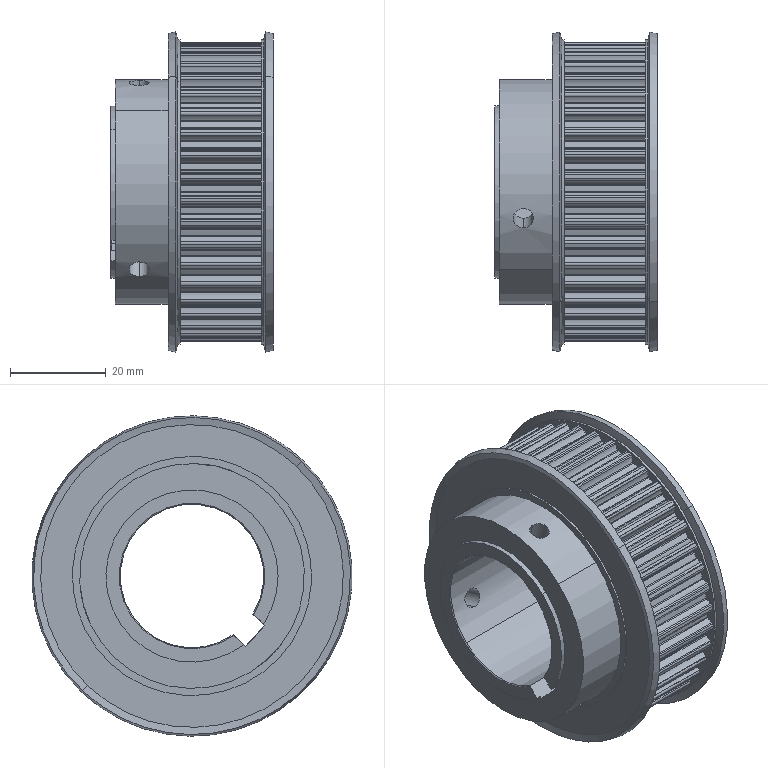Component | SolidWorks | HTPA40S5M150_B_H30-2 | 1 solid | 410 faces | box 34 x 67 x 67 mm | volume 60312 mm3 | cylinder 379 | cone 20 | plane 11 | commonest cylinder face diameters 1.1 x98 0.5 x92 6.55 x86 59.16 x41 62.7 x40 4.2 x6 50 x4 63.66 x4 | material 45#
build123d program:
from build123d import *

# Parameters (mm, degrees)
SKETCH2_W          = 127.32
SKETCH2_H          = 127.32
CUT_EXTRUDE1_DEPTH = 17
SKETCH3_W          = 6
SKETCH3_H          = 8.588
CUT_EXTRUDE2_DEPTH = 59.314
CIRPATTERN1_COUNT  = 3
SKETCH7_OUTSIDE_W  = 89.134
SKETCH7_OUTSIDE_H  = 89.134
SKETCH7_OUTSIDE_R  = 18
CUT_EXTRUDE3_DEPTH = 1


with BuildPart() as part:
    # Sketch1 → Revolve1 (revolve)
    with BuildSketch(Plane.XY, mode=Mode.PRIVATE) as revolve1_sk:
        Polygon((0, 24.8), (0, 15.2), (0.2, 15), (33.8, 15), (34, 15.2), (34, 23.3), (33.8, 23.5), (22, 23.5), (22, 25), (21.6, 25), (21.6, 31.641), (21.956, 33.127), (20.4, 33.5), (20, 31.83), (2, 31.83), (1.6, 33.5), (0.04401, 33.127), (0.4, 31.641), (0.4, 25), (0.2, 25), align=None)
    revolve(revolve1_sk.sketch.rotate(Axis((34, 0, 0), (-1, 0, 0)), 270), axis=Axis((34, 0, 0), (-1, 0, 0)))

    # Sketch2 → Cut-Extrude1 (cut)
    with BuildSketch(Plane(origin=(2.5, 0, 0), x_dir=(0, 0, -1), z_dir=(1, 0, 0))):
        Rectangle(SKETCH2_W, SKETCH2_H)
        with BuildLine():
            ThreePointArc((-31.28, 2.088), (-31.182, 1.735), (-30.884, 1.523))
            ThreePointArc((-30.884, 1.523), (-30.236, 1.259), (-29.66, 0.8639))
            ThreePointArc((-29.66, 0.8639), (-29.594, 0.7759), (-29.572, 0.6683))
            ThreePointArc((-29.572, 0.6683), (-29.58, 0), (-29.572, -0.6683))
            ThreePointArc((-29.572, -0.6683), (-29.594, -0.7759), (-29.66, -0.8639))
            ThreePointArc((-29.66, -0.8639), (-30.236, -1.259), (-30.884, -1.523))
            ThreePointArc((-30.884, -1.523), (-31.182, -1.735), (-31.28, -2.088))
            ThreePointArc((-31.28, -2.088), (-31.267, -2.274), (-31.253, -2.46))
            ThreePointArc((-31.253, -2.46), (-31.238, -2.646), (-31.222, -2.831))
            ThreePointArc((-31.222, -2.831), (-31.069, -3.164), (-30.742, -3.327))
            ThreePointArc((-30.742, -3.327), (-30.061, -3.487), (-29.43, -3.787))
            ThreePointArc((-29.43, -3.787), (-29.351, -3.863), (-29.313, -3.966))
            ThreePointArc((-29.313, -3.966), (-29.216, -4.627), (-29.104, -5.286))
            ThreePointArc((-29.104, -5.286), (-29.108, -5.396), (-29.16, -5.493))
            ThreePointArc((-29.16, -5.493), (-29.667, -5.973), (-30.265, -6.335))
            ThreePointArc((-30.265, -6.335), (-30.526, -6.592), (-30.569, -6.955))
            ThreePointArc((-30.569, -6.955), (-30.527, -7.137), (-30.484, -7.319))
            ThreePointArc((-30.484, -7.319), (-30.44, -7.5), (-30.395, -7.681))
            ThreePointArc((-30.395, -7.681), (-30.192, -7.986), (-29.843, -8.096))
            ThreePointArc((-29.843, -8.096), (-29.146, -8.146), (-28.475, -8.344))
            ThreePointArc((-28.475, -8.344), (-28.385, -8.407), (-28.332, -8.503))
            ThreePointArc((-28.332, -8.503), (-28.132, -9.141), (-27.919, -9.774))
            ThreePointArc((-27.919, -9.774), (-27.906, -9.883), (-27.941, -9.987))
            ThreePointArc((-27.941, -9.987), (-28.368, -10.541), (-28.902, -10.992))
            ThreePointArc((-28.902, -10.992), (-29.119, -11.286), (-29.104, -11.652))
            ThreePointArc((-29.104, -11.652), (-29.034, -11.825), (-28.964, -11.997))
            ThreePointArc((-28.964, -11.997), (-28.892, -12.169), (-28.819, -12.341))
            ThreePointArc((-28.819, -12.341), (-28.571, -12.61), (-28.209, -12.664))
            ThreePointArc((-28.209, -12.664), (-27.512, -12.605), (-26.819, -12.696))
            ThreePointArc((-26.819, -12.696), (-26.721, -12.744), (-26.653, -12.83))
            ThreePointArc((-26.653, -12.83), (-26.356, -13.429), (-26.046, -14.021))
            ThreePointArc((-26.046, -14.021), (-26.016, -14.127), (-26.035, -14.235))
            ThreePointArc((-26.035, -14.235), (-26.369, -14.849), (-26.826, -15.377))
            ThreePointArc((-26.826, -15.377), (-26.995, -15.702), (-26.923, -16.061))
            ThreePointArc((-26.923, -16.061), (-26.827, -16.221), (-26.73, -16.38))
            ThreePointArc((-26.73, -16.38), (-26.632, -16.539), (-26.534, -16.697))
            ThreePointArc((-26.534, -16.697), (-26.246, -16.924), (-25.88, -16.921))
            ThreePointArc((-25.88, -16.921), (-25.202, -16.754), (-24.503, -16.735))
            ThreePointArc((-24.503, -16.735), (-24.398, -16.767), (-24.317, -16.842))
            ThreePointArc((-24.317, -16.842), (-23.931, -17.387), (-23.532, -17.923))
            ThreePointArc((-23.532, -17.923), (-23.486, -18.023), (-23.488, -18.133))
            ThreePointArc((-23.488, -18.133), (-23.722, -18.791), (-24.09, -19.385))
            ThreePointArc((-24.09, -19.385), (-24.207, -19.732), (-24.079, -20.075))
            ThreePointArc((-24.079, -20.075), (-23.959, -20.218), (-23.839, -20.36))
            ThreePointArc((-23.839, -20.36), (-23.717, -20.502), (-23.595, -20.642))
            ThreePointArc((-23.595, -20.642), (-23.276, -20.822), (-22.915, -20.761))
            ThreePointArc((-22.915, -20.761), (-22.271, -20.49), (-21.584, -20.362))
            ThreePointArc((-21.584, -20.362), (-21.475, -20.378), (-21.383, -20.438))
            ThreePointArc((-21.383, -20.438), (-20.916, -20.916), (-20.438, -21.383))
            ThreePointArc((-20.438, -21.383), (-20.378, -21.475), (-20.362, -21.584))
            ThreePointArc((-20.362, -21.584), (-20.49, -22.271), (-20.761, -22.915))
            ThreePointArc((-20.761, -22.915), (-20.822, -23.276), (-20.642, -23.595))
            ThreePointArc((-20.642, -23.595), (-20.502, -23.717), (-20.36, -23.839))
            ThreePointArc((-20.36, -23.839), (-20.218, -23.959), (-20.075, -24.079))
            ThreePointArc((-20.075, -24.079), (-19.732, -24.207), (-19.385, -24.09))
            ThreePointArc((-19.385, -24.09), (-18.791, -23.722), (-18.133, -23.488))
            ThreePointArc((-18.133, -23.488), (-18.023, -23.486), (-17.923, -23.532))
            ThreePointArc((-17.923, -23.532), (-17.387, -23.931), (-16.842, -24.317))
            ThreePointArc((-16.842, -24.317), (-16.767, -24.398), (-16.735, -24.503))
            ThreePointArc((-16.735, -24.503), (-16.754, -25.202), (-16.921, -25.88))
            ThreePointArc((-16.921, -25.88), (-16.924, -26.246), (-16.697, -26.534))
            ThreePointArc((-16.697, -26.534), (-16.539, -26.632), (-16.38, -26.73))
            ThreePointArc((-16.38, -26.73), (-16.221, -26.827), (-16.061, -26.923))
            ThreePointArc((-16.061, -26.923), (-15.702, -26.995), (-15.377, -26.826))
            ThreePointArc((-15.377, -26.826), (-14.849, -26.369), (-14.235, -26.035))
            ThreePointArc((-14.235, -26.035), (-14.127, -26.016), (-14.021, -26.046))
            ThreePointArc((-14.021, -26.046), (-13.429, -26.356), (-12.83, -26.653))
            ThreePointArc((-12.83, -26.653), (-12.744, -26.721), (-12.696, -26.819))
            ThreePointArc((-12.696, -26.819), (-12.605, -27.512), (-12.664, -28.209))
            ThreePointArc((-12.664, -28.209), (-12.61, -28.571), (-12.341, -28.819))
            ThreePointArc((-12.341, -28.819), (-12.169, -28.892), (-11.997, -28.964))
            ThreePointArc((-11.997, -28.964), (-11.825, -29.034), (-11.652, -29.104))
            ThreePointArc((-11.652, -29.104), (-11.286, -29.119), (-10.992, -28.902))
            ThreePointArc((-10.992, -28.902), (-10.541, -28.368), (-9.987, -27.941))
            ThreePointArc((-9.987, -27.941), (-9.883, -27.906), (-9.774, -27.919))
            ThreePointArc((-9.774, -27.919), (-9.141, -28.132), (-8.503, -28.332))
            ThreePointArc((-8.503, -28.332), (-8.407, -28.385), (-8.344, -28.475))
            ThreePointArc((-8.344, -28.475), (-8.146, -29.146), (-8.096, -29.843))
            ThreePointArc((-8.096, -29.843), (-7.986, -30.192), (-7.681, -30.395))
            ThreePointArc((-7.681, -30.395), (-7.5, -30.44), (-7.319, -30.484))
            ThreePointArc((-7.319, -30.484), (-7.137, -30.527), (-6.955, -30.569))
            ThreePointArc((-6.955, -30.569), (-6.592, -30.526), (-6.335, -30.265))
            ThreePointArc((-6.335, -30.265), (-5.973, -29.667), (-5.493, -29.16))
            ThreePointArc((-5.493, -29.16), (-5.396, -29.108), (-5.286, -29.104))
            ThreePointArc((-5.286, -29.104), (-4.627, -29.216), (-3.966, -29.313))
            ThreePointArc((-3.966, -29.313), (-3.863, -29.351), (-3.787, -29.43))
            ThreePointArc((-3.787, -29.43), (-3.487, -30.061), (-3.327, -30.742))
            ThreePointArc((-3.327, -30.742), (-3.164, -31.069), (-2.831, -31.222))
            ThreePointArc((-2.831, -31.222), (-2.646, -31.238), (-2.46, -31.253))
            ThreePointArc((-2.46, -31.253), (-2.274, -31.267), (-2.088, -31.28))
            ThreePointArc((-2.088, -31.28), (-1.735, -31.182), (-1.523, -30.884))
            ThreePointArc((-1.523, -30.884), (-1.259, -30.236), (-0.8639, -29.66))
            ThreePointArc((-0.8639, -29.66), (-0.7759, -29.594), (-0.6683, -29.572))
            ThreePointArc((-0.6683, -29.572), (0, -29.58), (0.6683, -29.572))
            ThreePointArc((0.6683, -29.572), (0.7759, -29.594), (0.8639, -29.66))
            ThreePointArc((0.8639, -29.66), (1.259, -30.236), (1.523, -30.884))
            ThreePointArc((1.523, -30.884), (1.735, -31.182), (2.088, -31.28))
            ThreePointArc((2.088, -31.28), (2.274, -31.267), (2.46, -31.253))
            ThreePointArc((2.46, -31.253), (2.646, -31.238), (2.831, -31.222))
            ThreePointArc((2.831, -31.222), (3.164, -31.069), (3.327, -30.742))
            ThreePointArc((3.327, -30.742), (3.487, -30.061), (3.787, -29.43))
            ThreePointArc((3.787, -29.43), (3.863, -29.351), (3.966, -29.313))
            ThreePointArc((3.966, -29.313), (4.627, -29.216), (5.286, -29.104))
            ThreePointArc((5.286, -29.104), (5.396, -29.108), (5.493, -29.16))
            ThreePointArc((5.493, -29.16), (5.973, -29.667), (6.335, -30.265))
            ThreePointArc((6.335, -30.265), (6.592, -30.526), (6.955, -30.569))
            ThreePointArc((6.955, -30.569), (7.137, -30.527), (7.319, -30.484))
            ThreePointArc((7.319, -30.484), (7.5, -30.44), (7.681, -30.395))
            ThreePointArc((7.681, -30.395), (7.986, -30.192), (8.096, -29.843))
            ThreePointArc((8.096, -29.843), (8.146, -29.146), (8.344, -28.475))
            ThreePointArc((8.344, -28.475), (8.407, -28.385), (8.503, -28.332))
            ThreePointArc((8.503, -28.332), (9.141, -28.132), (9.774, -27.919))
            ThreePointArc((9.774, -27.919), (9.883, -27.906), (9.987, -27.941))
            ThreePointArc((9.987, -27.941), (10.541, -28.368), (10.992, -28.902))
            ThreePointArc((10.992, -28.902), (11.286, -29.119), (11.652, -29.104))
            ThreePointArc((11.652, -29.104), (11.825, -29.034), (11.997, -28.964))
            ThreePointArc((11.997, -28.964), (12.169, -28.892), (12.341, -28.819))
            ThreePointArc((12.341, -28.819), (12.61, -28.571), (12.664, -28.209))
            ThreePointArc((12.664, -28.209), (12.605, -27.512), (12.696, -26.819))
            ThreePointArc((12.696, -26.819), (12.744, -26.721), (12.83, -26.653))
            ThreePointArc((12.83, -26.653), (13.429, -26.356), (14.021, -26.046))
            ThreePointArc((14.021, -26.046), (14.127, -26.016), (14.235, -26.035))
            ThreePointArc((14.235, -26.035), (14.849, -26.369), (15.377, -26.826))
            ThreePointArc((15.377, -26.826), (15.702, -26.995), (16.061, -26.923))
            ThreePointArc((16.061, -26.923), (16.221, -26.827), (16.38, -26.73))
            ThreePointArc((16.38, -26.73), (16.539, -26.632), (16.697, -26.534))
            ThreePointArc((16.697, -26.534), (16.924, -26.246), (16.921, -25.88))
            ThreePointArc((16.921, -25.88), (16.754, -25.202), (16.735, -24.503))
            ThreePointArc((16.735, -24.503), (16.767, -24.398), (16.842, -24.317))
            ThreePointArc((16.842, -24.317), (17.387, -23.931), (17.923, -23.532))
            ThreePointArc((17.923, -23.532), (18.023, -23.486), (18.133, -23.488))
            ThreePointArc((18.133, -23.488), (18.791, -23.722), (19.385, -24.09))
            ThreePointArc((19.385, -24.09), (19.732, -24.207), (20.075, -24.079))
            ThreePointArc((20.075, -24.079), (20.218, -23.959), (20.36, -23.839))
            ThreePointArc((20.36, -23.839), (20.502, -23.717), (20.642, -23.595))
            ThreePointArc((20.642, -23.595), (20.822, -23.276), (20.761, -22.915))
            ThreePointArc((20.761, -22.915), (20.49, -22.271), (20.362, -21.584))
            ThreePointArc((20.362, -21.584), (20.378, -21.475), (20.438, -21.383))
            ThreePointArc((20.438, -21.383), (20.916, -20.916), (21.383, -20.438))
            ThreePointArc((21.383, -20.438), (21.475, -20.378), (21.584, -20.362))
            ThreePointArc((21.584, -20.362), (22.271, -20.49), (22.915, -20.761))
            ThreePointArc((22.915, -20.761), (23.276, -20.822), (23.595, -20.642))
            ThreePointArc((23.595, -20.642), (23.717, -20.502), (23.839, -20.36))
            ThreePointArc((23.839, -20.36), (23.959, -20.218), (24.079, -20.075))
            ThreePointArc((24.079, -20.075), (24.207, -19.732), (24.09, -19.385))
            ThreePointArc((24.09, -19.385), (23.722, -18.791), (23.488, -18.133))
            ThreePointArc((23.488, -18.133), (23.486, -18.023), (23.532, -17.923))
            ThreePointArc((23.532, -17.923), (23.931, -17.387), (24.317, -16.842))
            ThreePointArc((24.317, -16.842), (24.398, -16.767), (24.503, -16.735))
            ThreePointArc((24.503, -16.735), (25.202, -16.754), (25.88, -16.921))
            ThreePointArc((25.88, -16.921), (26.246, -16.924), (26.534, -16.697))
            ThreePointArc((26.534, -16.697), (26.632, -16.539), (26.73, -16.38))
            ThreePointArc((26.73, -16.38), (26.827, -16.221), (26.923, -16.061))
            ThreePointArc((26.923, -16.061), (26.995, -15.702), (26.826, -15.377))
            ThreePointArc((26.826, -15.377), (26.369, -14.849), (26.035, -14.235))
            ThreePointArc((26.035, -14.235), (26.016, -14.127), (26.046, -14.021))
            ThreePointArc((26.046, -14.021), (26.356, -13.429), (26.653, -12.83))
            ThreePointArc((26.653, -12.83), (26.721, -12.744), (26.819, -12.696))
            ThreePointArc((26.819, -12.696), (27.512, -12.605), (28.209, -12.664))
            ThreePointArc((28.209, -12.664), (28.571, -12.61), (28.819, -12.341))
            ThreePointArc((28.819, -12.341), (28.892, -12.169), (28.964, -11.997))
            ThreePointArc((28.964, -11.997), (29.034, -11.825), (29.104, -11.652))
            ThreePointArc((29.104, -11.652), (29.119, -11.286), (28.902, -10.992))
            ThreePointArc((28.902, -10.992), (28.368, -10.541), (27.941, -9.987))
            ThreePointArc((27.941, -9.987), (27.906, -9.883), (27.919, -9.774))
            ThreePointArc((27.919, -9.774), (28.132, -9.141), (28.332, -8.503))
            ThreePointArc((28.332, -8.503), (28.385, -8.407), (28.475, -8.344))
            ThreePointArc((28.475, -8.344), (29.146, -8.146), (29.843, -8.096))
            ThreePointArc((29.843, -8.096), (30.192, -7.986), (30.395, -7.681))
            ThreePointArc((30.395, -7.681), (30.44, -7.5), (30.484, -7.319))
            ThreePointArc((30.484, -7.319), (30.527, -7.137), (30.569, -6.955))
            ThreePointArc((30.569, -6.955), (30.526, -6.592), (30.265, -6.335))
            ThreePointArc((30.265, -6.335), (29.667, -5.973), (29.16, -5.493))
            ThreePointArc((29.16, -5.493), (29.108, -5.396), (29.104, -5.286))
            ThreePointArc((29.104, -5.286), (29.216, -4.627), (29.313, -3.966))
            ThreePointArc((29.313, -3.966), (29.351, -3.863), (29.43, -3.787))
            ThreePointArc((29.43, -3.787), (30.061, -3.487), (30.742, -3.327))
            ThreePointArc((30.742, -3.327), (31.069, -3.164), (31.222, -2.831))
            ThreePointArc((31.222, -2.831), (31.238, -2.646), (31.253, -2.46))
            ThreePointArc((31.253, -2.46), (31.267, -2.274), (31.28, -2.088))
            ThreePointArc((31.28, -2.088), (31.182, -1.735), (30.884, -1.523))
            ThreePointArc((30.884, -1.523), (30.236, -1.259), (29.66, -0.8639))
            ThreePointArc((29.66, -0.8639), (29.594, -0.7759), (29.572, -0.6683))
            ThreePointArc((29.572, -0.6683), (29.58, 0), (29.572, 0.6683))
            ThreePointArc((29.572, 0.6683), (29.594, 0.7759), (29.66, 0.8639))
            ThreePointArc((29.66, 0.8639), (30.236, 1.259), (30.884, 1.523))
            ThreePointArc((30.884, 1.523), (31.182, 1.735), (31.28, 2.088))
            ThreePointArc((31.28, 2.088), (31.267, 2.274), (31.253, 2.46))
            ThreePointArc((31.253, 2.46), (31.238, 2.646), (31.222, 2.831))
            ThreePointArc((31.222, 2.831), (31.069, 3.164), (30.742, 3.327))
            ThreePointArc((30.742, 3.327), (30.061, 3.487), (29.43, 3.787))
            ThreePointArc((29.43, 3.787), (29.351, 3.863), (29.313, 3.966))
            ThreePointArc((29.313, 3.966), (29.216, 4.627), (29.104, 5.286))
            ThreePointArc((29.104, 5.286), (29.108, 5.396), (29.16, 5.493))
            ThreePointArc((29.16, 5.493), (29.667, 5.973), (30.265, 6.335))
            ThreePointArc((30.265, 6.335), (30.526, 6.592), (30.569, 6.955))
            ThreePointArc((30.569, 6.955), (30.527, 7.137), (30.484, 7.319))
            ThreePointArc((30.484, 7.319), (30.44, 7.5), (30.395, 7.681))
            ThreePointArc((30.395, 7.681), (30.192, 7.986), (29.843, 8.096))
            ThreePointArc((29.843, 8.096), (29.146, 8.146), (28.475, 8.344))
            ThreePointArc((28.475, 8.344), (28.385, 8.407), (28.332, 8.503))
            ThreePointArc((28.332, 8.503), (28.132, 9.141), (27.919, 9.774))
            ThreePointArc((27.919, 9.774), (27.906, 9.883), (27.941, 9.987))
            ThreePointArc((27.941, 9.987), (28.368, 10.541), (28.902, 10.992))
            ThreePointArc((28.902, 10.992), (29.119, 11.286), (29.104, 11.652))
            ThreePointArc((29.104, 11.652), (29.034, 11.825), (28.964, 11.997))
            ThreePointArc((28.964, 11.997), (28.892, 12.169), (28.819, 12.341))
            ThreePointArc((28.819, 12.341), (28.571, 12.61), (28.209, 12.664))
            ThreePointArc((28.209, 12.664), (27.512, 12.605), (26.819, 12.696))
            ThreePointArc((26.819, 12.696), (26.721, 12.744), (26.653, 12.83))
            ThreePointArc((26.653, 12.83), (26.356, 13.429), (26.046, 14.021))
            ThreePointArc((26.046, 14.021), (26.016, 14.127), (26.035, 14.235))
            ThreePointArc((26.035, 14.235), (26.369, 14.849), (26.826, 15.377))
            ThreePointArc((26.826, 15.377), (26.995, 15.702), (26.923, 16.061))
            ThreePointArc((26.923, 16.061), (26.827, 16.221), (26.73, 16.38))
            ThreePointArc((26.73, 16.38), (26.632, 16.539), (26.534, 16.697))
            ThreePointArc((26.534, 16.697), (26.246, 16.924), (25.88, 16.921))
            ThreePointArc((25.88, 16.921), (25.202, 16.754), (24.503, 16.735))
            ThreePointArc((24.503, 16.735), (24.398, 16.767), (24.317, 16.842))
            ThreePointArc((24.317, 16.842), (23.931, 17.387), (23.532, 17.923))
            ThreePointArc((23.532, 17.923), (23.486, 18.023), (23.488, 18.133))
            ThreePointArc((23.488, 18.133), (23.722, 18.791), (24.09, 19.385))
            ThreePointArc((24.09, 19.385), (24.207, 19.732), (24.079, 20.075))
            ThreePointArc((24.079, 20.075), (23.959, 20.218), (23.839, 20.36))
            ThreePointArc((23.839, 20.36), (23.717, 20.502), (23.595, 20.642))
            ThreePointArc((23.595, 20.642), (23.276, 20.822), (22.915, 20.761))
            ThreePointArc((22.915, 20.761), (22.271, 20.49), (21.584, 20.362))
            ThreePointArc((21.584, 20.362), (21.475, 20.378), (21.383, 20.438))
            ThreePointArc((21.383, 20.438), (20.916, 20.916), (20.438, 21.383))
            ThreePointArc((20.438, 21.383), (20.378, 21.475), (20.362, 21.584))
            ThreePointArc((20.362, 21.584), (20.49, 22.271), (20.761, 22.915))
            ThreePointArc((20.761, 22.915), (20.822, 23.276), (20.642, 23.595))
            ThreePointArc((20.642, 23.595), (20.502, 23.717), (20.36, 23.839))
            ThreePointArc((20.36, 23.839), (20.218, 23.959), (20.075, 24.079))
            ThreePointArc((20.075, 24.079), (19.732, 24.207), (19.385, 24.09))
            ThreePointArc((19.385, 24.09), (18.791, 23.722), (18.133, 23.488))
            ThreePointArc((18.133, 23.488), (18.023, 23.486), (17.923, 23.532))
            ThreePointArc((17.923, 23.532), (17.387, 23.931), (16.842, 24.317))
            ThreePointArc((16.842, 24.317), (16.767, 24.398), (16.735, 24.503))
            ThreePointArc((16.735, 24.503), (16.754, 25.202), (16.921, 25.88))
            ThreePointArc((16.921, 25.88), (16.924, 26.246), (16.697, 26.534))
            ThreePointArc((16.697, 26.534), (16.539, 26.632), (16.38, 26.73))
            ThreePointArc((16.38, 26.73), (16.221, 26.827), (16.061, 26.923))
            ThreePointArc((16.061, 26.923), (15.702, 26.995), (15.377, 26.826))
            ThreePointArc((15.377, 26.826), (14.849, 26.369), (14.235, 26.035))
            ThreePointArc((14.235, 26.035), (14.127, 26.016), (14.021, 26.046))
            ThreePointArc((14.021, 26.046), (13.429, 26.356), (12.83, 26.653))
            ThreePointArc((12.83, 26.653), (12.744, 26.721), (12.696, 26.819))
            ThreePointArc((12.696, 26.819), (12.605, 27.512), (12.664, 28.209))
            ThreePointArc((12.664, 28.209), (12.61, 28.571), (12.341, 28.819))
            ThreePointArc((12.341, 28.819), (12.169, 28.892), (11.997, 28.964))
            ThreePointArc((11.997, 28.964), (11.825, 29.034), (11.652, 29.104))
            ThreePointArc((11.652, 29.104), (11.286, 29.119), (10.992, 28.902))
            ThreePointArc((10.992, 28.902), (10.541, 28.368), (9.987, 27.941))
            ThreePointArc((9.987, 27.941), (9.883, 27.906), (9.774, 27.919))
            ThreePointArc((9.774, 27.919), (9.141, 28.132), (8.503, 28.332))
            ThreePointArc((8.503, 28.332), (8.407, 28.385), (8.344, 28.475))
            ThreePointArc((8.344, 28.475), (8.146, 29.146), (8.096, 29.843))
            ThreePointArc((8.096, 29.843), (7.986, 30.192), (7.681, 30.395))
            ThreePointArc((7.681, 30.395), (7.5, 30.44), (7.319, 30.484))
            ThreePointArc((7.319, 30.484), (7.137, 30.527), (6.955, 30.569))
            ThreePointArc((6.955, 30.569), (6.592, 30.526), (6.335, 30.265))
            ThreePointArc((6.335, 30.265), (5.973, 29.667), (5.493, 29.16))
            ThreePointArc((5.493, 29.16), (5.396, 29.108), (5.286, 29.104))
            ThreePointArc((5.286, 29.104), (4.627, 29.216), (3.966, 29.313))
            ThreePointArc((3.966, 29.313), (3.863, 29.351), (3.787, 29.43))
            ThreePointArc((3.787, 29.43), (3.487, 30.061), (3.327, 30.742))
            ThreePointArc((3.327, 30.742), (3.164, 31.069), (2.831, 31.222))
            ThreePointArc((2.831, 31.222), (2.646, 31.238), (2.46, 31.253))
            ThreePointArc((2.46, 31.253), (2.274, 31.267), (2.088, 31.28))
            ThreePointArc((2.088, 31.28), (1.735, 31.182), (1.523, 30.884))
            ThreePointArc((1.523, 30.884), (1.259, 30.236), (0.8639, 29.66))
            ThreePointArc((0.8639, 29.66), (0.7759, 29.594), (0.6683, 29.572))
            ThreePointArc((0.6683, 29.572), (0, 29.58), (-0.6683, 29.572))
            ThreePointArc((-0.6683, 29.572), (-0.7759, 29.594), (-0.8639, 29.66))
            ThreePointArc((-0.8639, 29.66), (-1.259, 30.236), (-1.523, 30.884))
            ThreePointArc((-1.523, 30.884), (-1.735, 31.182), (-2.088, 31.28))
            ThreePointArc((-2.088, 31.28), (-2.274, 31.267), (-2.46, 31.253))
            ThreePointArc((-2.46, 31.253), (-2.646, 31.238), (-2.831, 31.222))
            ThreePointArc((-2.831, 31.222), (-3.164, 31.069), (-3.327, 30.742))
            ThreePointArc((-3.327, 30.742), (-3.487, 30.061), (-3.787, 29.43))
            ThreePointArc((-3.787, 29.43), (-3.863, 29.351), (-3.966, 29.313))
            ThreePointArc((-3.966, 29.313), (-4.627, 29.216), (-5.286, 29.104))
            ThreePointArc((-5.286, 29.104), (-5.396, 29.108), (-5.493, 29.16))
            ThreePointArc((-5.493, 29.16), (-5.973, 29.667), (-6.335, 30.265))
            ThreePointArc((-6.335, 30.265), (-6.592, 30.526), (-6.955, 30.569))
            ThreePointArc((-6.955, 30.569), (-7.137, 30.527), (-7.319, 30.484))
            ThreePointArc((-7.319, 30.484), (-7.5, 30.44), (-7.681, 30.395))
            ThreePointArc((-7.681, 30.395), (-7.986, 30.192), (-8.096, 29.843))
            ThreePointArc((-8.096, 29.843), (-8.146, 29.146), (-8.344, 28.475))
            ThreePointArc((-8.344, 28.475), (-8.407, 28.385), (-8.503, 28.332))
            ThreePointArc((-8.503, 28.332), (-9.141, 28.132), (-9.774, 27.919))
            ThreePointArc((-9.774, 27.919), (-9.883, 27.906), (-9.987, 27.941))
            ThreePointArc((-9.987, 27.941), (-10.541, 28.368), (-10.992, 28.902))
            ThreePointArc((-10.992, 28.902), (-11.286, 29.119), (-11.652, 29.104))
            ThreePointArc((-11.652, 29.104), (-11.825, 29.034), (-11.997, 28.964))
            ThreePointArc((-11.997, 28.964), (-12.169, 28.892), (-12.341, 28.819))
            ThreePointArc((-12.341, 28.819), (-12.61, 28.571), (-12.664, 28.209))
            ThreePointArc((-12.664, 28.209), (-12.605, 27.512), (-12.696, 26.819))
            ThreePointArc((-12.696, 26.819), (-12.744, 26.721), (-12.83, 26.653))
            ThreePointArc((-12.83, 26.653), (-13.429, 26.356), (-14.021, 26.046))
            ThreePointArc((-14.021, 26.046), (-14.127, 26.016), (-14.235, 26.035))
            ThreePointArc((-14.235, 26.035), (-14.849, 26.369), (-15.377, 26.826))
            ThreePointArc((-15.377, 26.826), (-15.702, 26.995), (-16.061, 26.923))
            ThreePointArc((-16.061, 26.923), (-16.221, 26.827), (-16.38, 26.73))
            ThreePointArc((-16.38, 26.73), (-16.539, 26.632), (-16.697, 26.534))
            ThreePointArc((-16.697, 26.534), (-16.924, 26.246), (-16.921, 25.88))
            ThreePointArc((-16.921, 25.88), (-16.754, 25.202), (-16.735, 24.503))
            ThreePointArc((-16.735, 24.503), (-16.767, 24.398), (-16.842, 24.317))
            ThreePointArc((-16.842, 24.317), (-17.387, 23.931), (-17.923, 23.532))
            ThreePointArc((-17.923, 23.532), (-18.023, 23.486), (-18.133, 23.488))
            ThreePointArc((-18.133, 23.488), (-18.791, 23.722), (-19.385, 24.09))
            ThreePointArc((-19.385, 24.09), (-19.732, 24.207), (-20.075, 24.079))
            ThreePointArc((-20.075, 24.079), (-20.218, 23.959), (-20.36, 23.839))
            ThreePointArc((-20.36, 23.839), (-20.502, 23.717), (-20.642, 23.595))
            ThreePointArc((-20.642, 23.595), (-20.822, 23.276), (-20.761, 22.915))
            ThreePointArc((-20.761, 22.915), (-20.49, 22.271), (-20.362, 21.584))
            ThreePointArc((-20.362, 21.584), (-20.378, 21.475), (-20.438, 21.383))
            ThreePointArc((-20.438, 21.383), (-20.916, 20.916), (-21.383, 20.438))
            ThreePointArc((-21.383, 20.438), (-21.475, 20.378), (-21.584, 20.362))
            ThreePointArc((-21.584, 20.362), (-22.271, 20.49), (-22.915, 20.761))
            ThreePointArc((-22.915, 20.761), (-23.276, 20.822), (-23.595, 20.642))
            ThreePointArc((-23.595, 20.642), (-23.717, 20.502), (-23.839, 20.36))
            ThreePointArc((-23.839, 20.36), (-23.959, 20.218), (-24.079, 20.075))
            ThreePointArc((-24.079, 20.075), (-24.207, 19.732), (-24.09, 19.385))
            ThreePointArc((-24.09, 19.385), (-23.722, 18.791), (-23.488, 18.133))
            ThreePointArc((-23.488, 18.133), (-23.486, 18.023), (-23.532, 17.923))
            ThreePointArc((-23.532, 17.923), (-23.931, 17.387), (-24.317, 16.842))
            ThreePointArc((-24.317, 16.842), (-24.398, 16.767), (-24.503, 16.735))
            ThreePointArc((-24.503, 16.735), (-25.202, 16.754), (-25.88, 16.921))
            ThreePointArc((-25.88, 16.921), (-26.246, 16.924), (-26.534, 16.697))
            ThreePointArc((-26.534, 16.697), (-26.632, 16.539), (-26.73, 16.38))
            ThreePointArc((-26.73, 16.38), (-26.827, 16.221), (-26.923, 16.061))
            ThreePointArc((-26.923, 16.061), (-26.995, 15.702), (-26.826, 15.377))
            ThreePointArc((-26.826, 15.377), (-26.369, 14.849), (-26.035, 14.235))
            ThreePointArc((-26.035, 14.235), (-26.016, 14.127), (-26.046, 14.021))
            ThreePointArc((-26.046, 14.021), (-26.356, 13.429), (-26.653, 12.83))
            ThreePointArc((-26.653, 12.83), (-26.721, 12.744), (-26.819, 12.696))
            ThreePointArc((-26.819, 12.696), (-27.512, 12.605), (-28.209, 12.664))
            ThreePointArc((-28.209, 12.664), (-28.571, 12.61), (-28.819, 12.341))
            ThreePointArc((-28.819, 12.341), (-28.892, 12.169), (-28.964, 11.997))
            ThreePointArc((-28.964, 11.997), (-29.034, 11.825), (-29.104, 11.652))
            ThreePointArc((-29.104, 11.652), (-29.119, 11.286), (-28.902, 10.992))
            ThreePointArc((-28.902, 10.992), (-28.368, 10.541), (-27.941, 9.987))
            ThreePointArc((-27.941, 9.987), (-27.906, 9.883), (-27.919, 9.774))
            ThreePointArc((-27.919, 9.774), (-28.132, 9.141), (-28.332, 8.503))
            ThreePointArc((-28.332, 8.503), (-28.385, 8.407), (-28.475, 8.344))
            ThreePointArc((-28.475, 8.344), (-29.146, 8.146), (-29.843, 8.096))
            ThreePointArc((-29.843, 8.096), (-30.192, 7.986), (-30.395, 7.681))
            ThreePointArc((-30.395, 7.681), (-30.44, 7.5), (-30.484, 7.319))
            ThreePointArc((-30.484, 7.319), (-30.527, 7.137), (-30.569, 6.955))
            ThreePointArc((-30.569, 6.955), (-30.526, 6.592), (-30.265, 6.335))
            ThreePointArc((-30.265, 6.335), (-29.667, 5.973), (-29.16, 5.493))
            ThreePointArc((-29.16, 5.493), (-29.108, 5.396), (-29.104, 5.286))
            ThreePointArc((-29.104, 5.286), (-29.216, 4.627), (-29.313, 3.966))
            ThreePointArc((-29.313, 3.966), (-29.351, 3.863), (-29.43, 3.787))
            ThreePointArc((-29.43, 3.787), (-30.061, 3.487), (-30.742, 3.327))
            ThreePointArc((-30.742, 3.327), (-31.069, 3.164), (-31.222, 2.831))
            ThreePointArc((-31.222, 2.831), (-31.238, 2.646), (-31.253, 2.46))
            ThreePointArc((-31.253, 2.46), (-31.267, 2.274), (-31.28, 2.088))
        make_face(mode=Mode.SUBTRACT)
    extrude(amount=CUT_EXTRUDE1_DEPTH, mode=Mode.SUBTRACT)

    # Sketch3 → Cut-Extrude2 (cut, through all)
    with BuildSketch(Plane(origin=(34, 0, 0), x_dir=(0, 0, -1), z_dir=(1, 0, 0))):
        with Locations((0, 13.906)):
            Rectangle(SKETCH3_W, SKETCH3_H)
    extrude(amount=-CUT_EXTRUDE2_DEPTH, mode=Mode.SUBTRACT)

    # Sketch6 → M5 Tapped Hole1 (revolve, cut)
    with BuildSketch(Plane(origin=(28, 0, 0), x_dir=(0, 0, -1), z_dir=(1, 0, 0))):
        Polygon((0, 0), (0, 45.762), (2.1, 45.762), (2.1, 0.425), (2.525, 0), align=None)
    m5_tapped_hole1 = revolve(axis=Axis((28, -6.35, 0), (0, 1, 0)), mode=Mode.SUBTRACT)

    # CirPattern1: M5 Tapped Hole1 ×3 about axis
    cirpattern1_axis = Axis((33.8, 0, 0), (-1, 0, 0))
    for i in range(1, CIRPATTERN1_COUNT):
        add(m5_tapped_hole1.rotate(cirpattern1_axis, i * 360 / CIRPATTERN1_COUNT), mode=Mode.SUBTRACT)

    # Sketch7 outside → Cut-Extrude3 (cut)
    with BuildSketch(Plane(origin=(34, 0, 0), x_dir=(0, 0, -1), z_dir=(1, 0, 0))):
        Rectangle(SKETCH7_OUTSIDE_W, SKETCH7_OUTSIDE_H)
        Circle(SKETCH7_OUTSIDE_R, mode=Mode.SUBTRACT)
    extrude(amount=-CUT_EXTRUDE3_DEPTH, mode=Mode.SUBTRACT)


solid = part.part

# Placed as in the assembly
solid = solid.moved(Location((32.41, -29.263, -16.52), (43.558, 0, -180)))